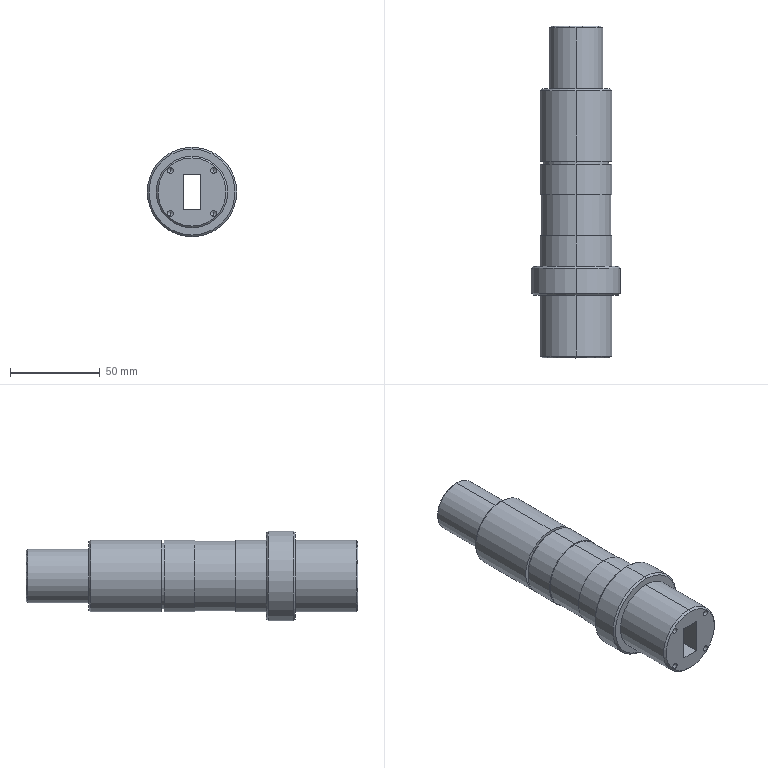Component | SolidWorks | BearingHousingAssembly-1_BuckleRotaryAxis-1 | 1 solid | 55 faces | box 50 x 185 x 50 mm | volume 184981 mm3 | cylinder 24 | cone 18 | plane 13 | commonest cylinder face diameters 3.3 x8 40 x8 30 x2 39 x2 36.5 x2 50 x2
build123d program:
from build123d import *

# Parameters (mm, degrees)
SKETCH1_R           = 20
BOSS_EXTRUDE1_DEPTH = 150
SKETCH2_W           = 20
SKETCH2_H           = 10
CUT_EXTRUDE1_DEPTH  = 153.643
SKETCH4_W           = 1.6
SKETCH4_H           = 1.75
SKETCH5_R           = 25
SKETCH5_R_2         = 13.416
BOSS_EXTRUDE2_DEPTH = 51
SKETCH6_R           = 25
SKETCH6_R_2         = 20
CUT_EXTRUDE3_DEPTH  = 35
CHAMFER2_SIZE       = 1
CIRPATTERN1_COUNT   = 4
SKETCH9_W           = 23
SKETCH9_H           = 10.212
SKETCH10_R          = 15
SKETCH10_W          = 20
SKETCH10_H          = 10
BOSS_EXTRUDE3_DEPTH = 35
CHAMFER3_SIZE       = 1


with BuildPart() as part:
    # Sketch1 → Boss-Extrude1 (new body)
    with BuildSketch(Plane.XY):
        Circle(SKETCH1_R)
    extrude(amount=BOSS_EXTRUDE1_DEPTH)

    # Sketch2 → Cut-Extrude1 (cut, through all)
    with BuildSketch(Plane.XY.offset(150)):
        Rectangle(SKETCH2_W, SKETCH2_H)
    extrude(amount=-CUT_EXTRUDE1_DEPTH, mode=Mode.SUBTRACT)

    # Sketch4 → Cut-Revolve1 (revolve, cut)
    with BuildSketch(Plane(origin=(0, 0, 0), x_dir=(0, 0, -1), z_dir=(1, 0, 0)), mode=Mode.PRIVATE) as cut_revolve1_sk:
        with Locations((-108.8, 19.125)):
            Rectangle(SKETCH4_W, SKETCH4_H)
    revolve(cut_revolve1_sk.sketch.rotate(Axis((0, 0, 0), (0, 0, 1)), 90), axis=Axis((0, 0, 0), (0, 0, 1)), mode=Mode.SUBTRACT)

    # Sketch5 → Boss-Extrude2 (add)
    with BuildSketch(Plane(origin=(0, 0, 0), x_dir=(-1, 0, 0), z_dir=(0, 0, -1))):
        Circle(SKETCH5_R)
        Circle(SKETCH5_R_2, mode=Mode.SUBTRACT)
    extrude(amount=-BOSS_EXTRUDE2_DEPTH)

    # Sketch6 → Cut-Extrude3 (cut)
    with BuildSketch(Plane(origin=(0, 0, 0), x_dir=(-1, 0, 0), z_dir=(0, 0, -1))):
        Circle(SKETCH6_R)
        Circle(SKETCH6_R_2, mode=Mode.SUBTRACT)
    extrude(amount=-CUT_EXTRUDE3_DEPTH, mode=Mode.SUBTRACT)

    # Sketch7 → M4 Tapped Hole1 (revolve, cut)
    with BuildSketch(Plane(origin=(-12.021, 12.021, 0), x_dir=(0, 1, 0), z_dir=(1, 0, 0))):
        Polygon((0, 0), (0, 14.591), (1.65, 13.6), (1.65, 0), align=None)
    m4_tapped_hole1 = revolve(axis=Axis((-12.021, 12.021, -6.35), (0, 0, 1)), mode=Mode.SUBTRACT)

    # Chamfer2
    chamfer2_edges = [part.edges().sort_by_distance(p)[0] for p in [
        (25, 0, 51),
        (25, 0, 35),
        (20, 0, 0),
        (-20, 0, 150),
    ]]
    chamfer(chamfer2_edges, length=CHAMFER2_SIZE)

    # CirPattern1: M4 Tapped Hole1 ×4 about axis
    cirpattern1_axis = Axis((0, 0, 0), (0, 0, 1))
    for i in range(1, CIRPATTERN1_COUNT):
        add(m4_tapped_hole1.rotate(cirpattern1_axis, i * 360 / CIRPATTERN1_COUNT), mode=Mode.SUBTRACT)

    # Sketch9 → Cut-Revolve2 (revolve, cut)
    with BuildSketch(Plane(origin=(0, 0, 0), x_dir=(0, 0, -1), z_dir=(1, 0, 0)), mode=Mode.PRIVATE) as cut_revolve2_sk:
        with Locations((-79.5, -24.606)):
            Rectangle(SKETCH9_W, SKETCH9_H)
    revolve(cut_revolve2_sk.sketch.rotate(Axis((0, 0, 0), (0, 0, 1)), 270), axis=Axis((0, 0, 0), (0, 0, 1)), mode=Mode.SUBTRACT)

    # Sketch10 → Boss-Extrude3 (add)
    with BuildSketch(Plane.XY.offset(150)):
        Circle(SKETCH10_R)
        Rectangle(SKETCH10_W, SKETCH10_H, mode=Mode.SUBTRACT)
    extrude(amount=BOSS_EXTRUDE3_DEPTH)

    # Chamfer3
    chamfer3_edges = [part.edges().sort_by_distance(p)[0] for p in [
        (-15, 0, 185),
    ]]
    chamfer(chamfer3_edges, length=CHAMFER3_SIZE)


solid = part.part

# Placed as in the assembly
solid = solid.moved(Location((-38.666, 129.264, -6), (-90, 0, 90)))